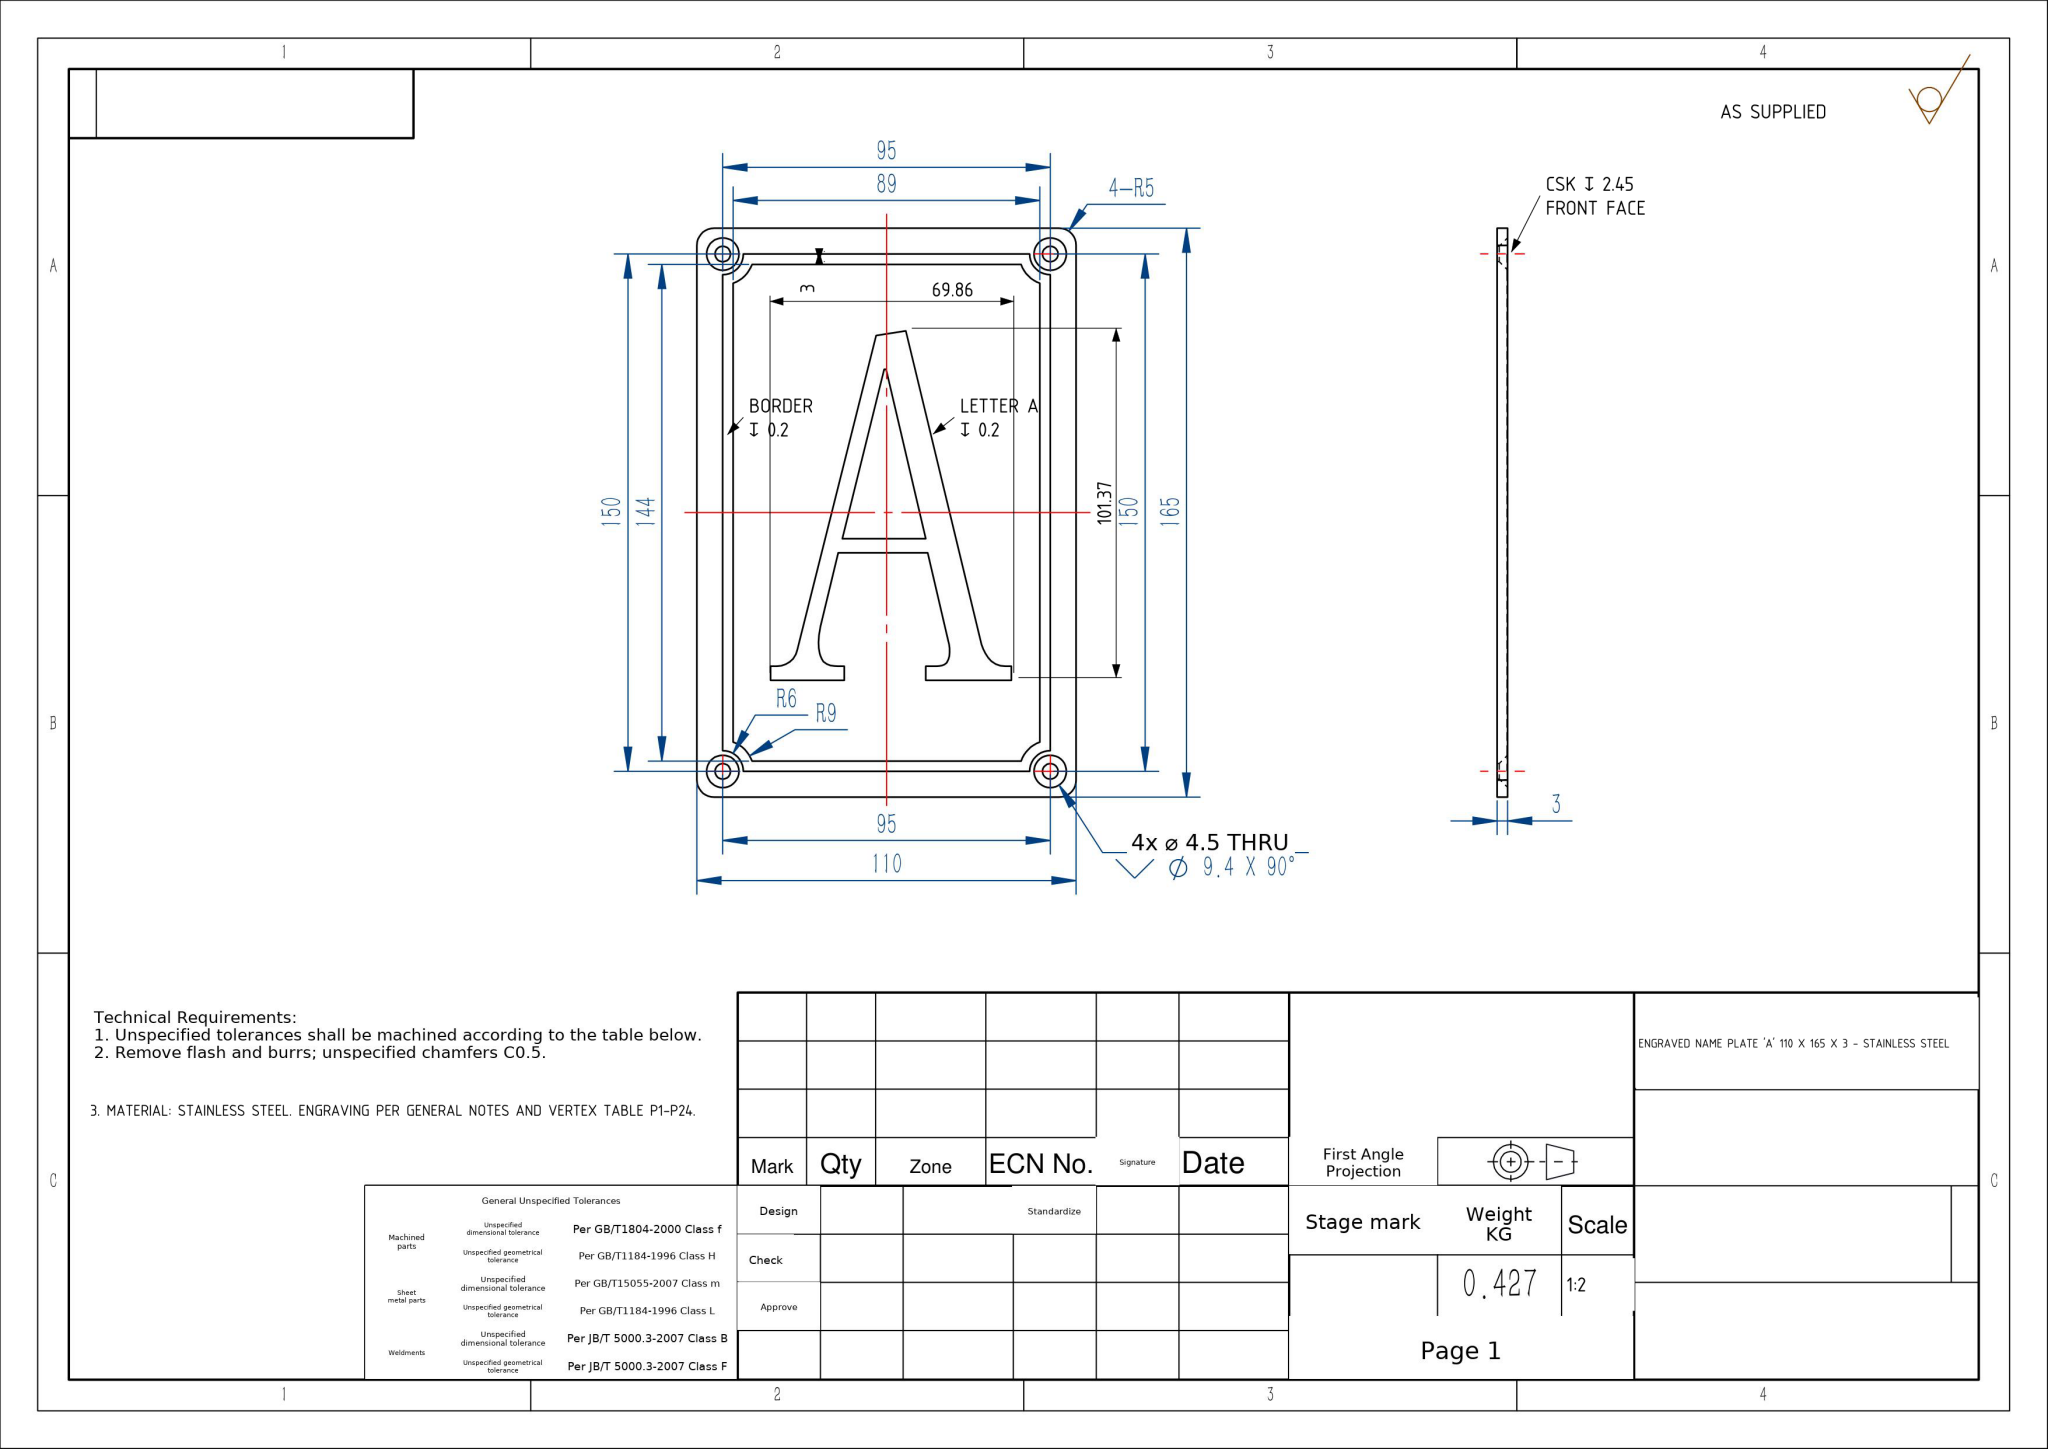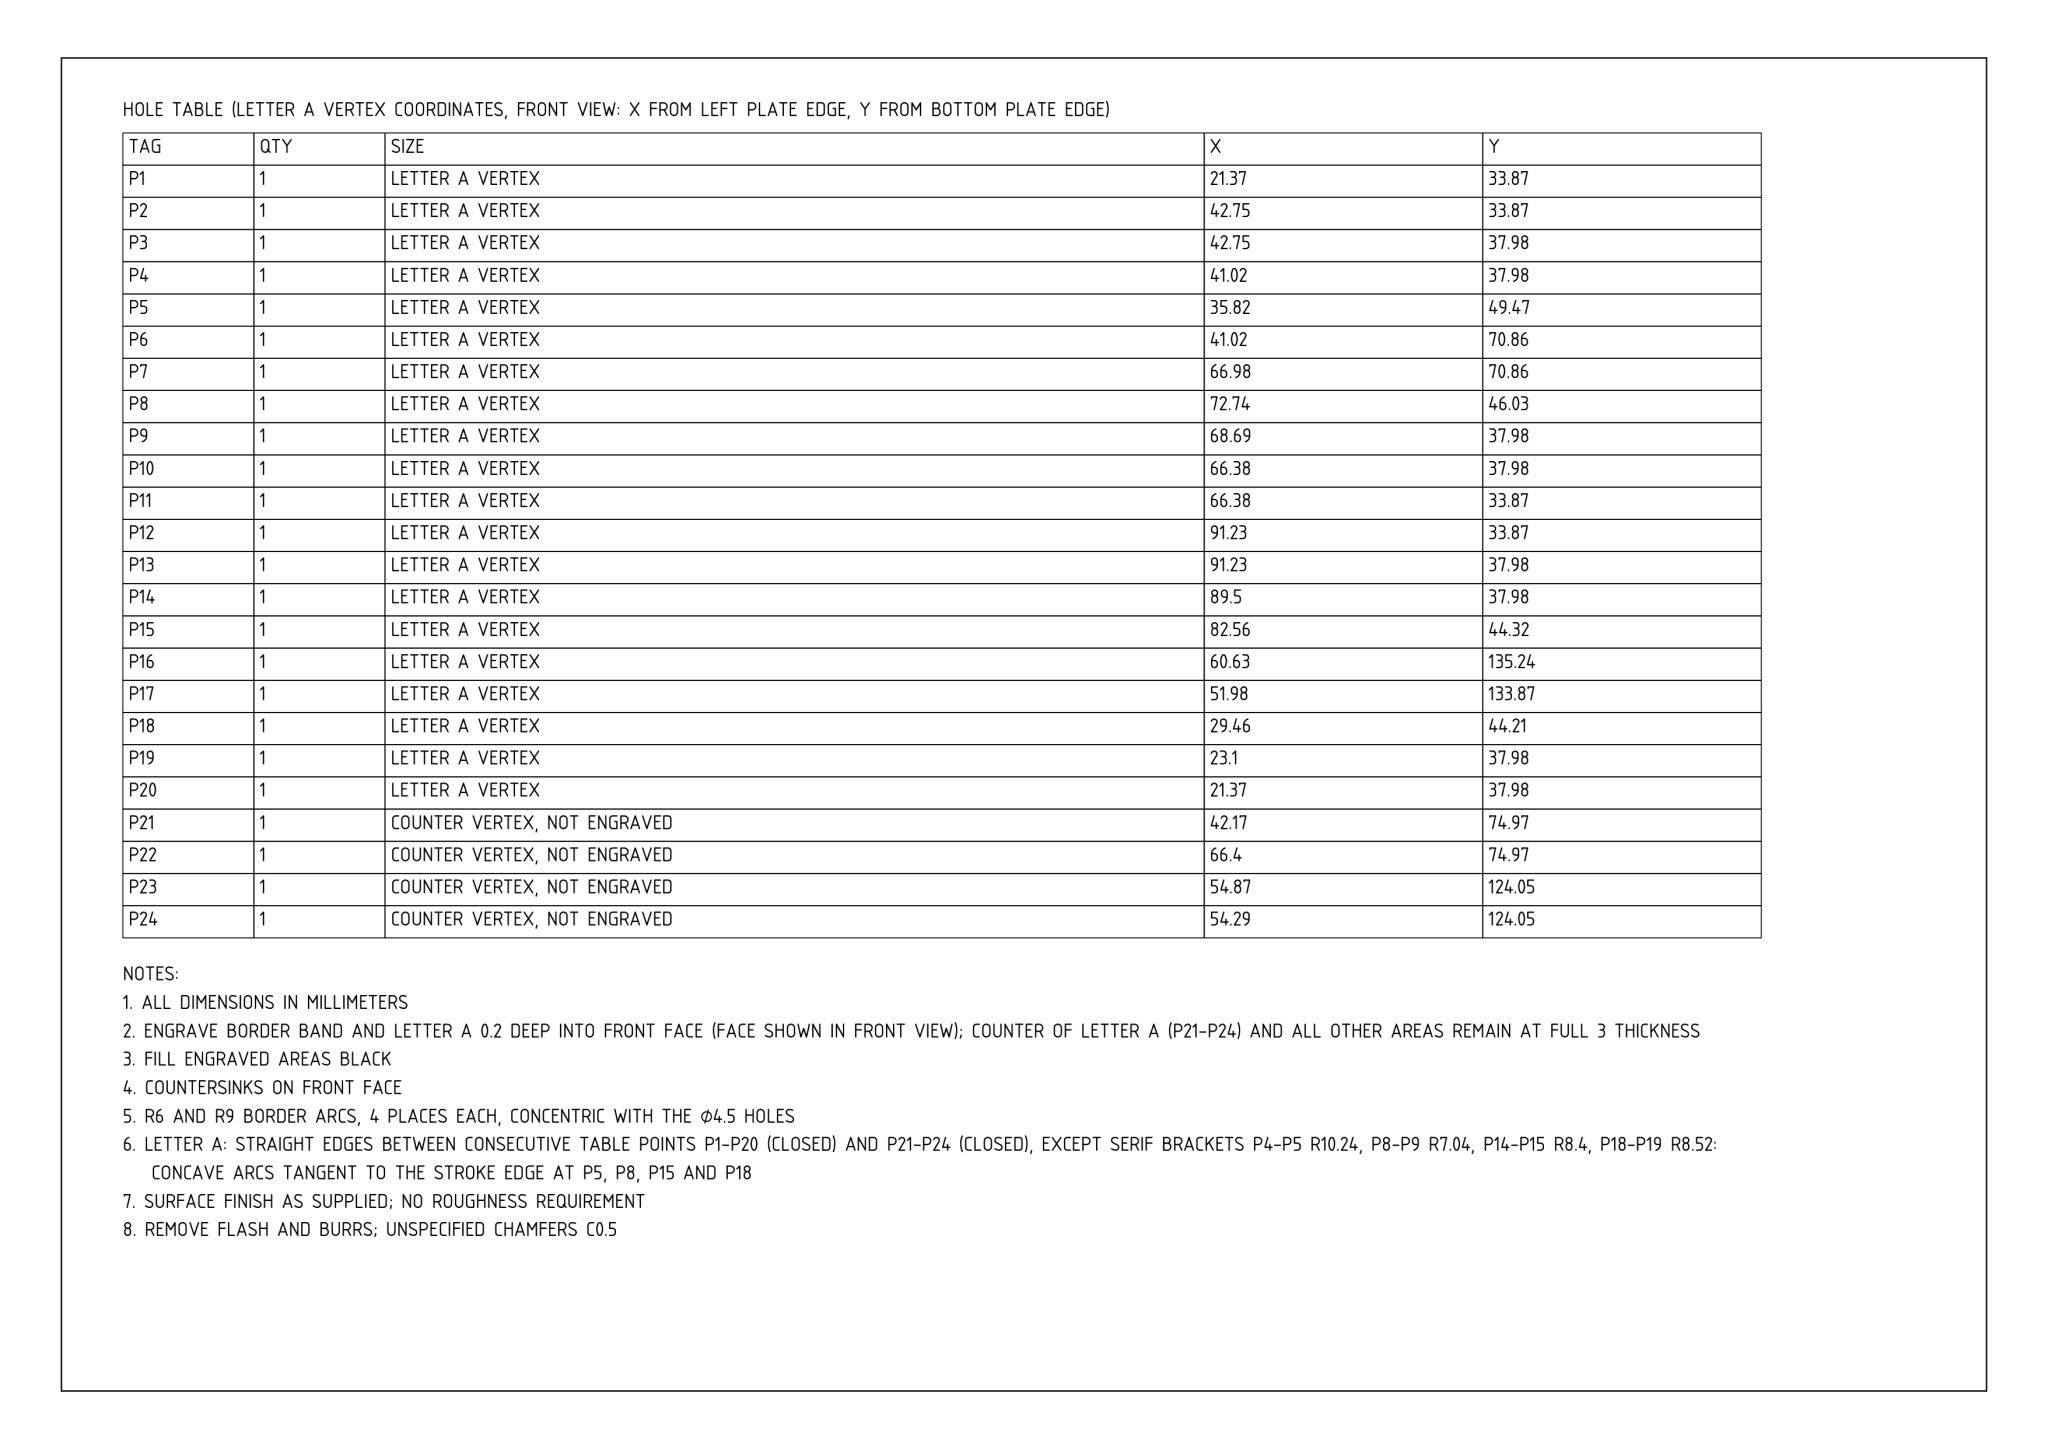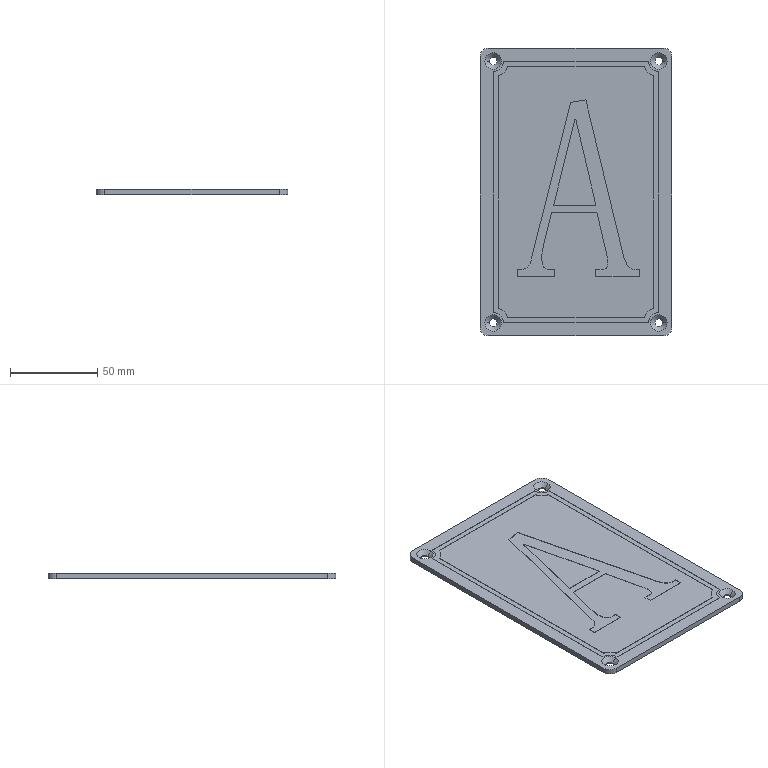Part | NX | mm | 1 solid | 72 faces | box 110 x 165 x 3 mm | volume 53357 mm3 | plane 38 | cylinder 20 | cone 8 | spline 6 | commonest cylinder face diameters 4.5 x8 12 x4 18 x4 10 x4